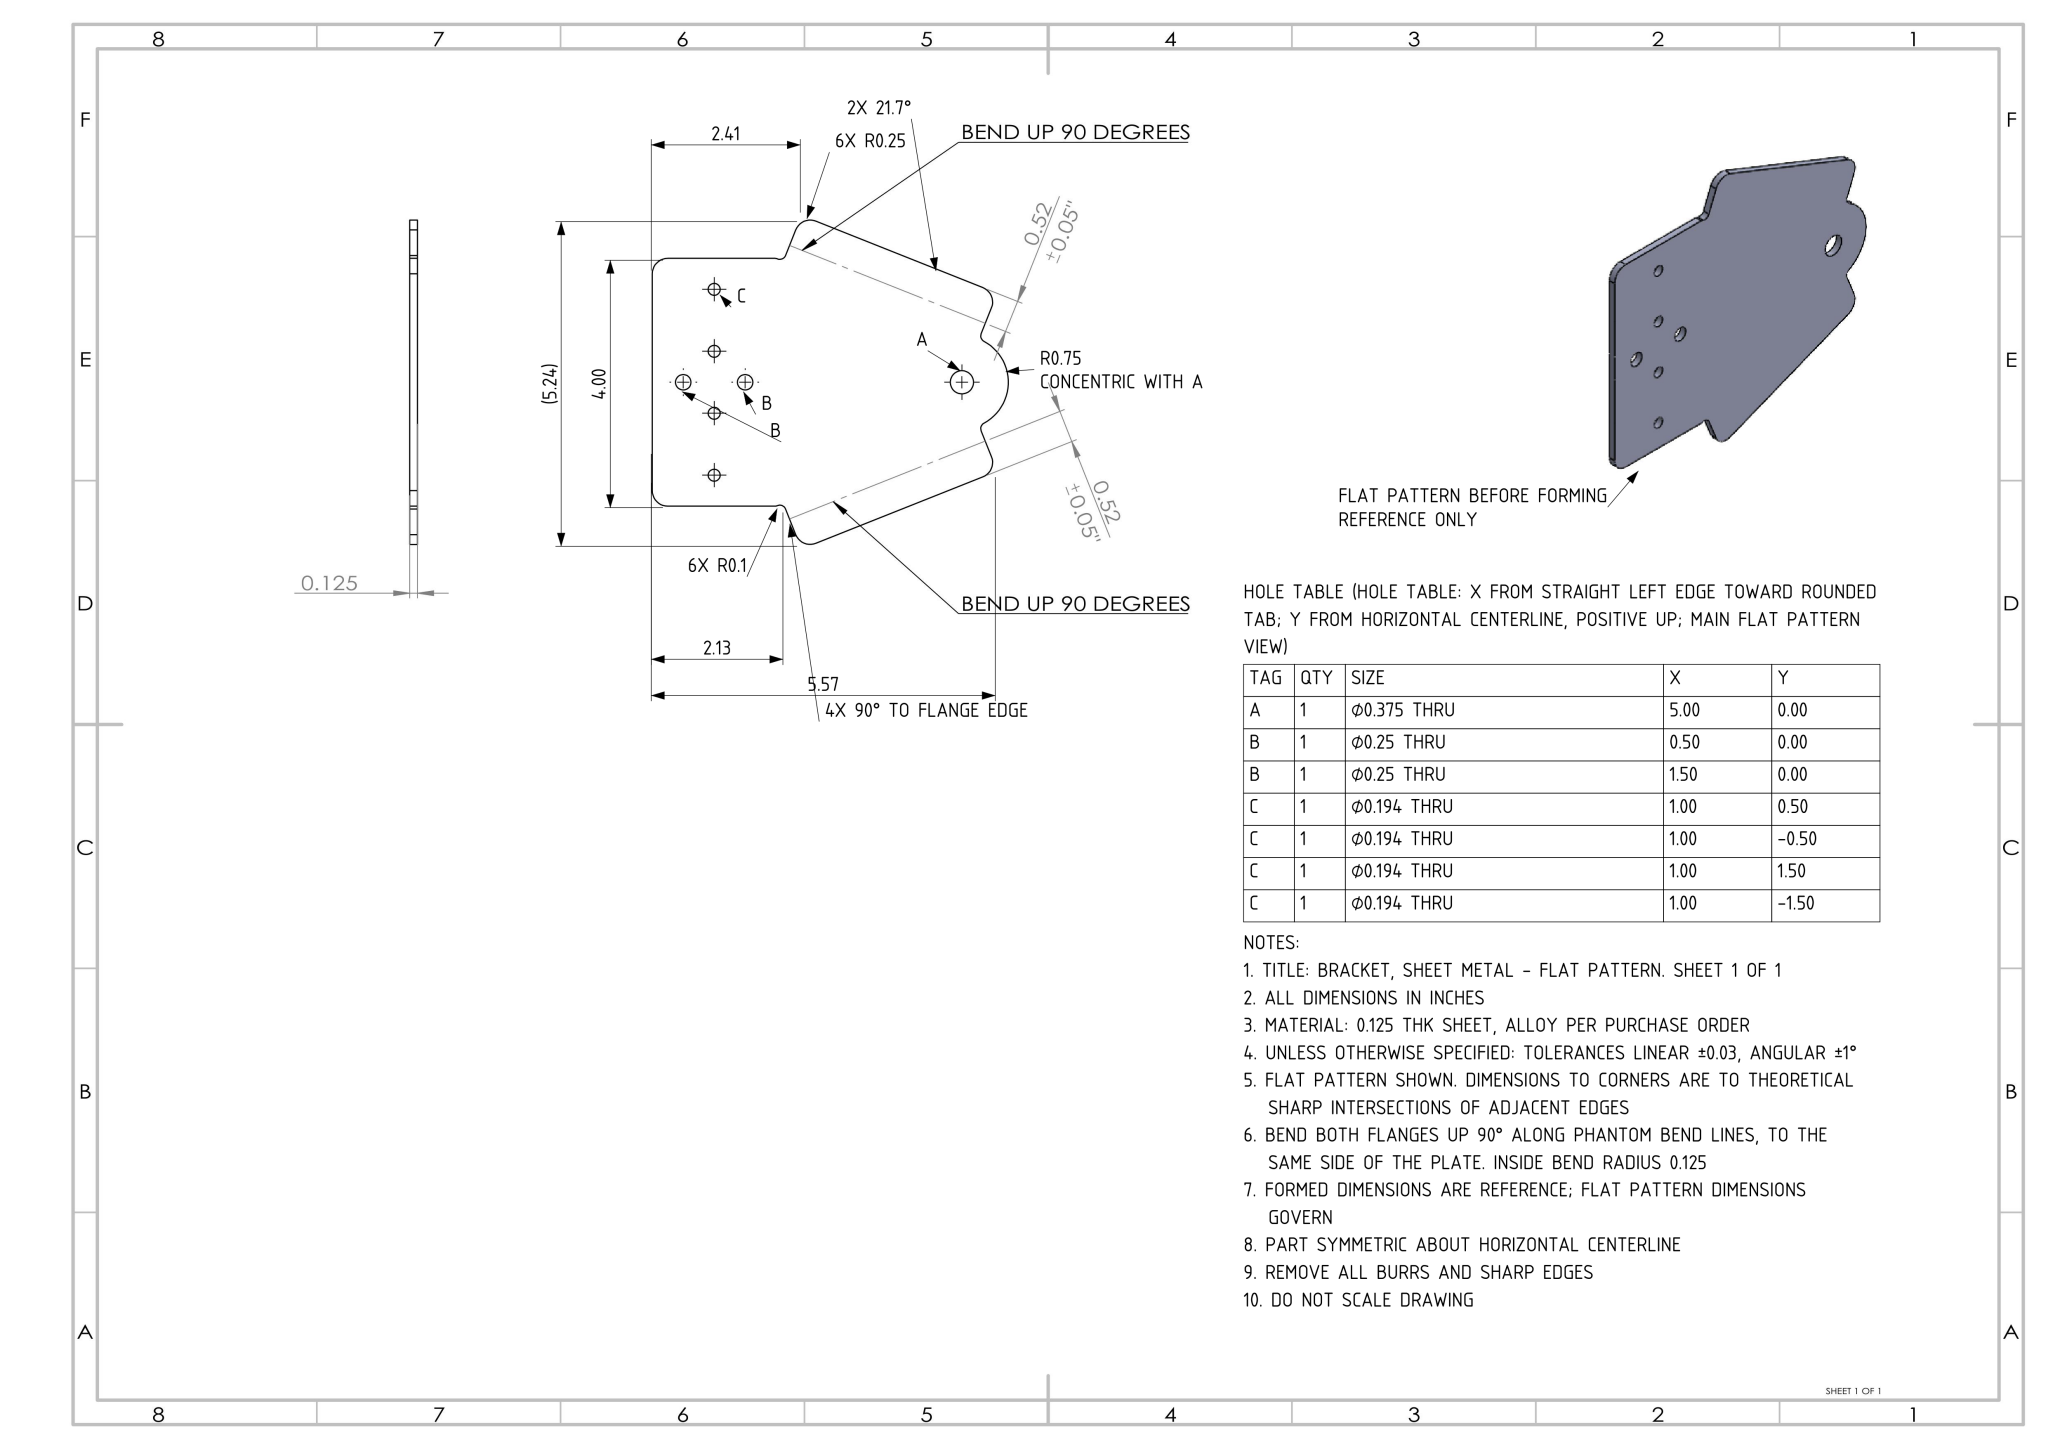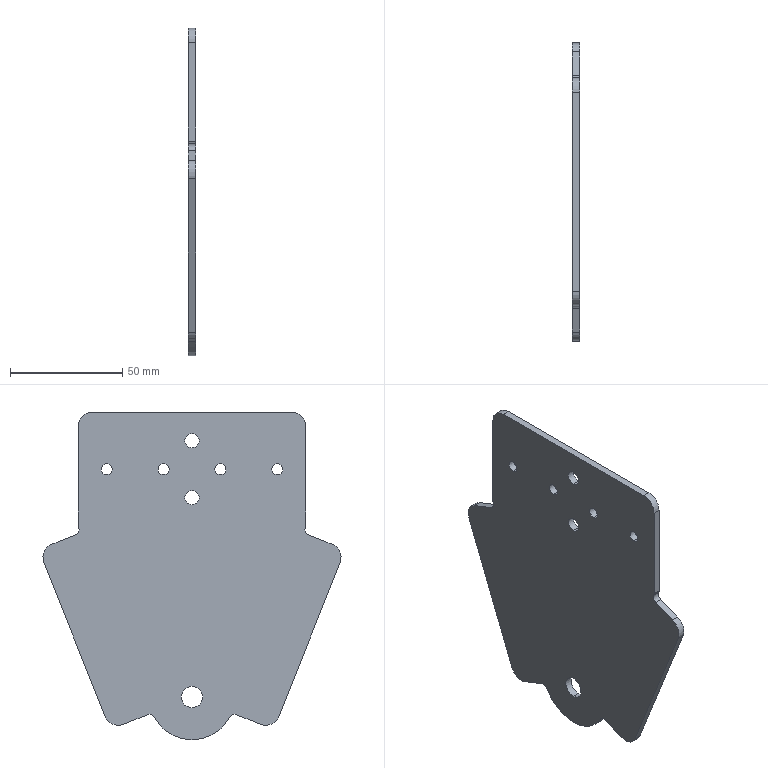Part | NX | drawing in inches | 1 solid | 41 faces | box 3.18 x 132.97 x 146.05 mm | volume 45723 mm3 | cylinder 28 | plane 13 | commonest cylinder face diameters 4.928 x8 12.7 x6 5.08 x6 6.35 x4 9.525 x2 38.1 x2